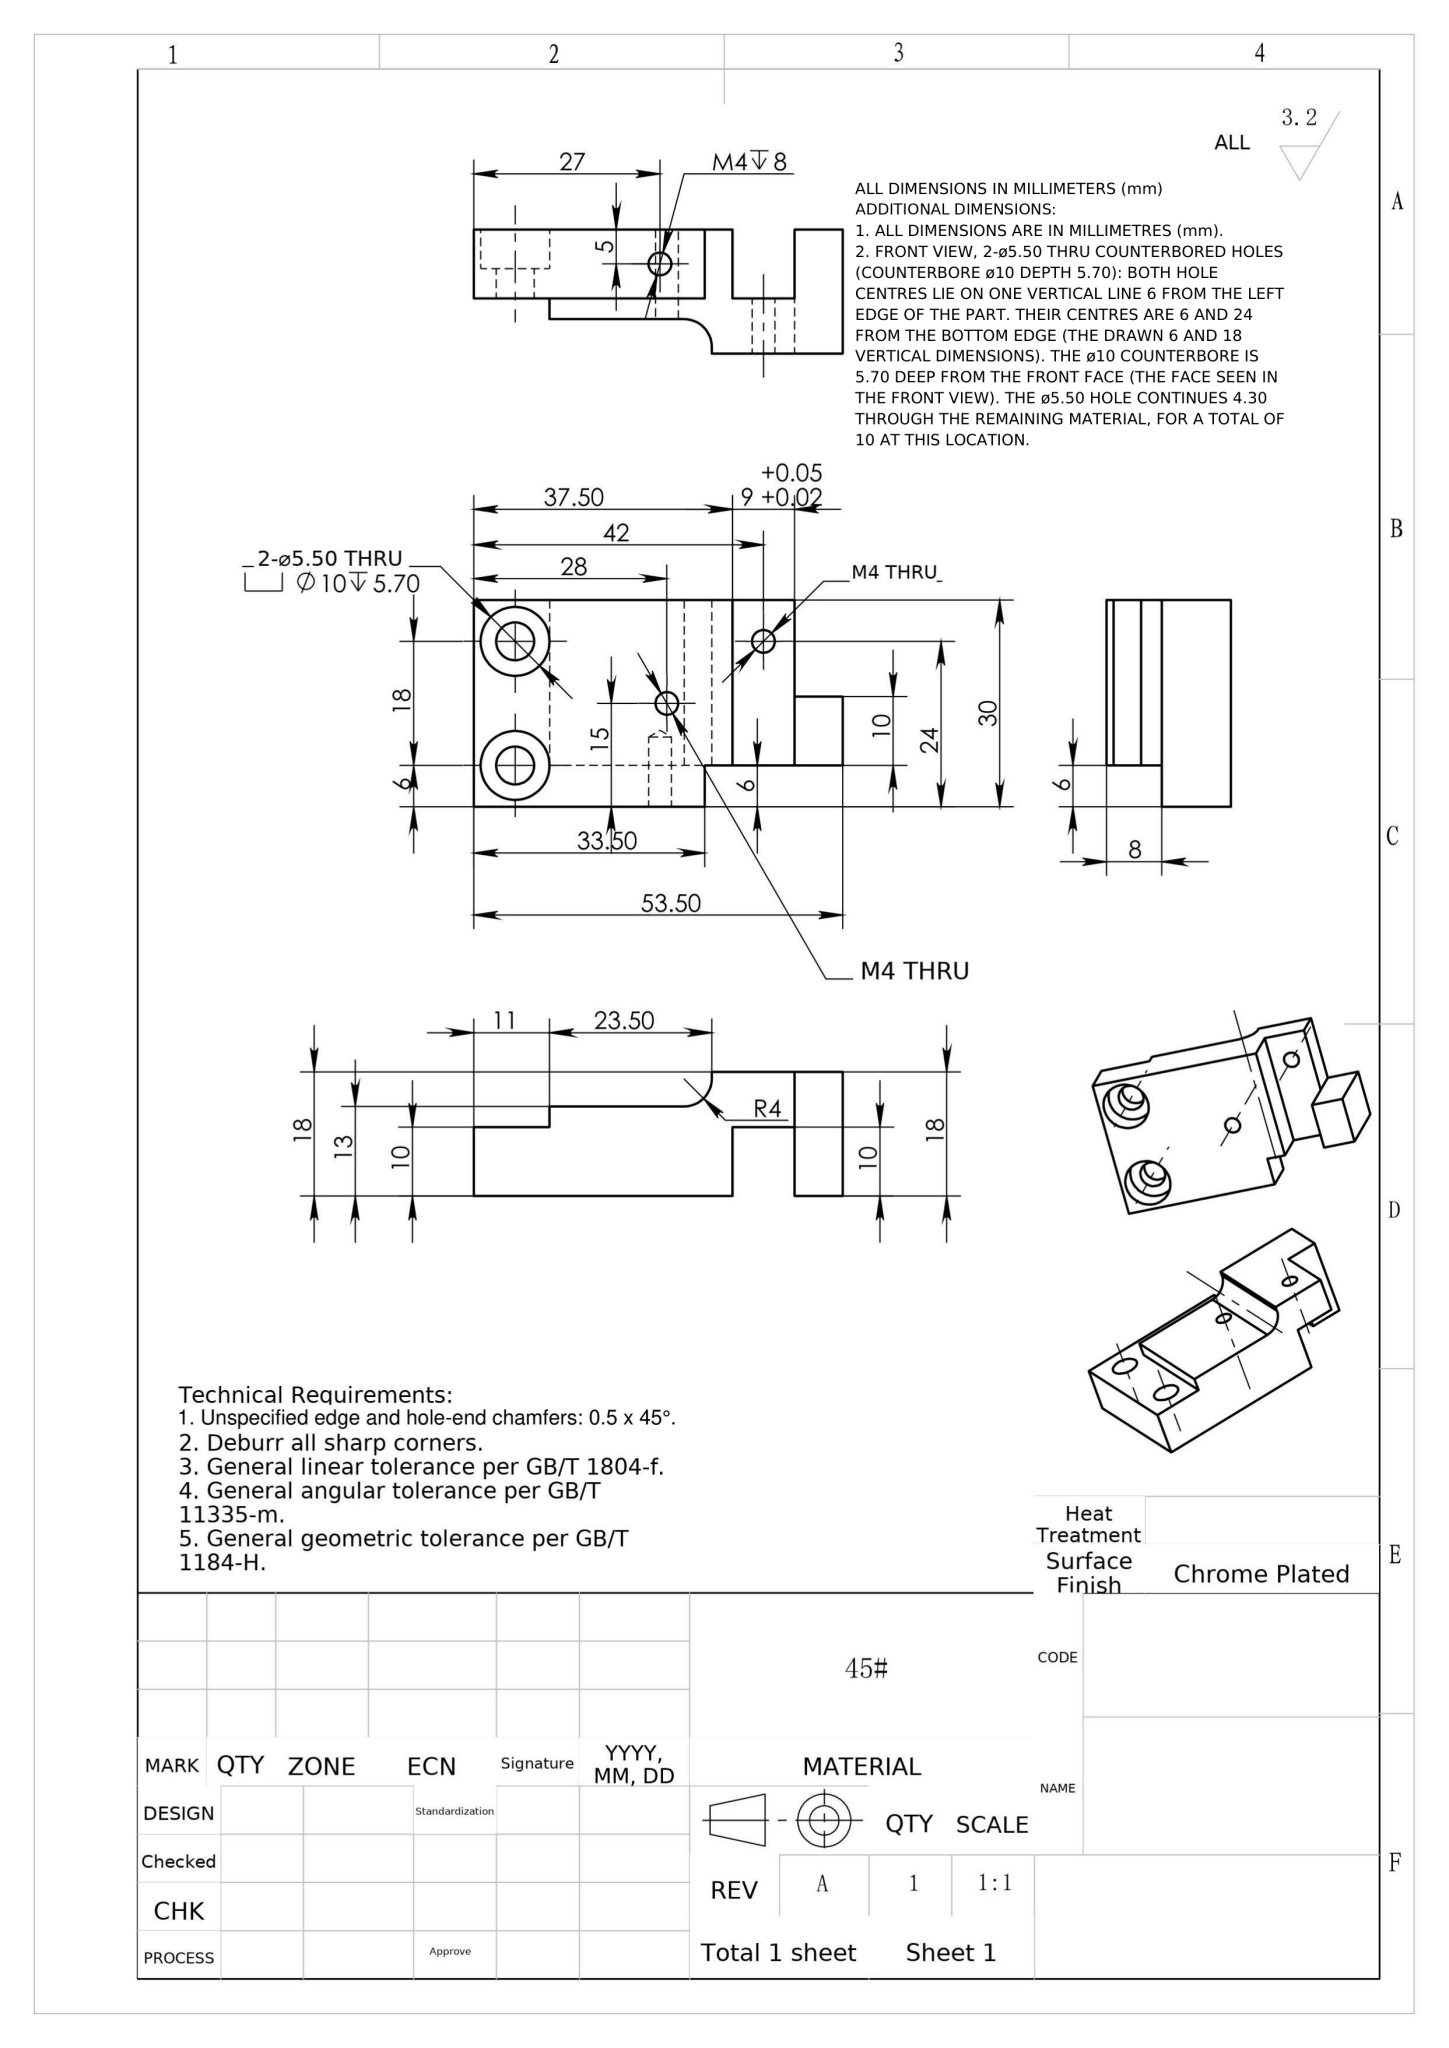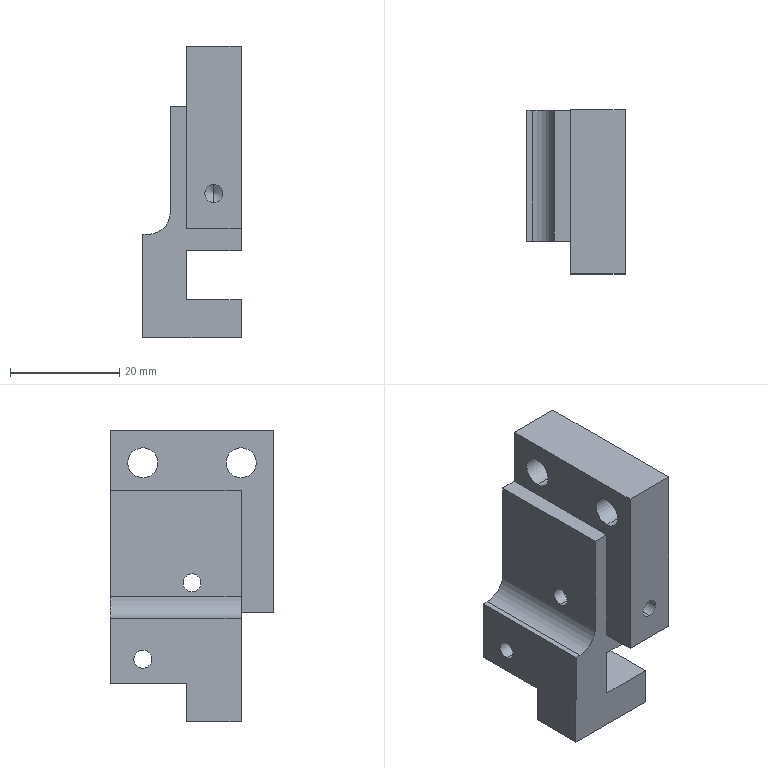Part | NX | mm | Stepped Multi-Bore L-Bracket | 1 solid | 37 faces | box 18 x 30 x 53.5 mm | volume 14980 mm3 | plane 20 | cylinder 15 | cone 2 | commonest cylinder face diameters 3.3 x6 10 x4 5.5 x4 8 x1